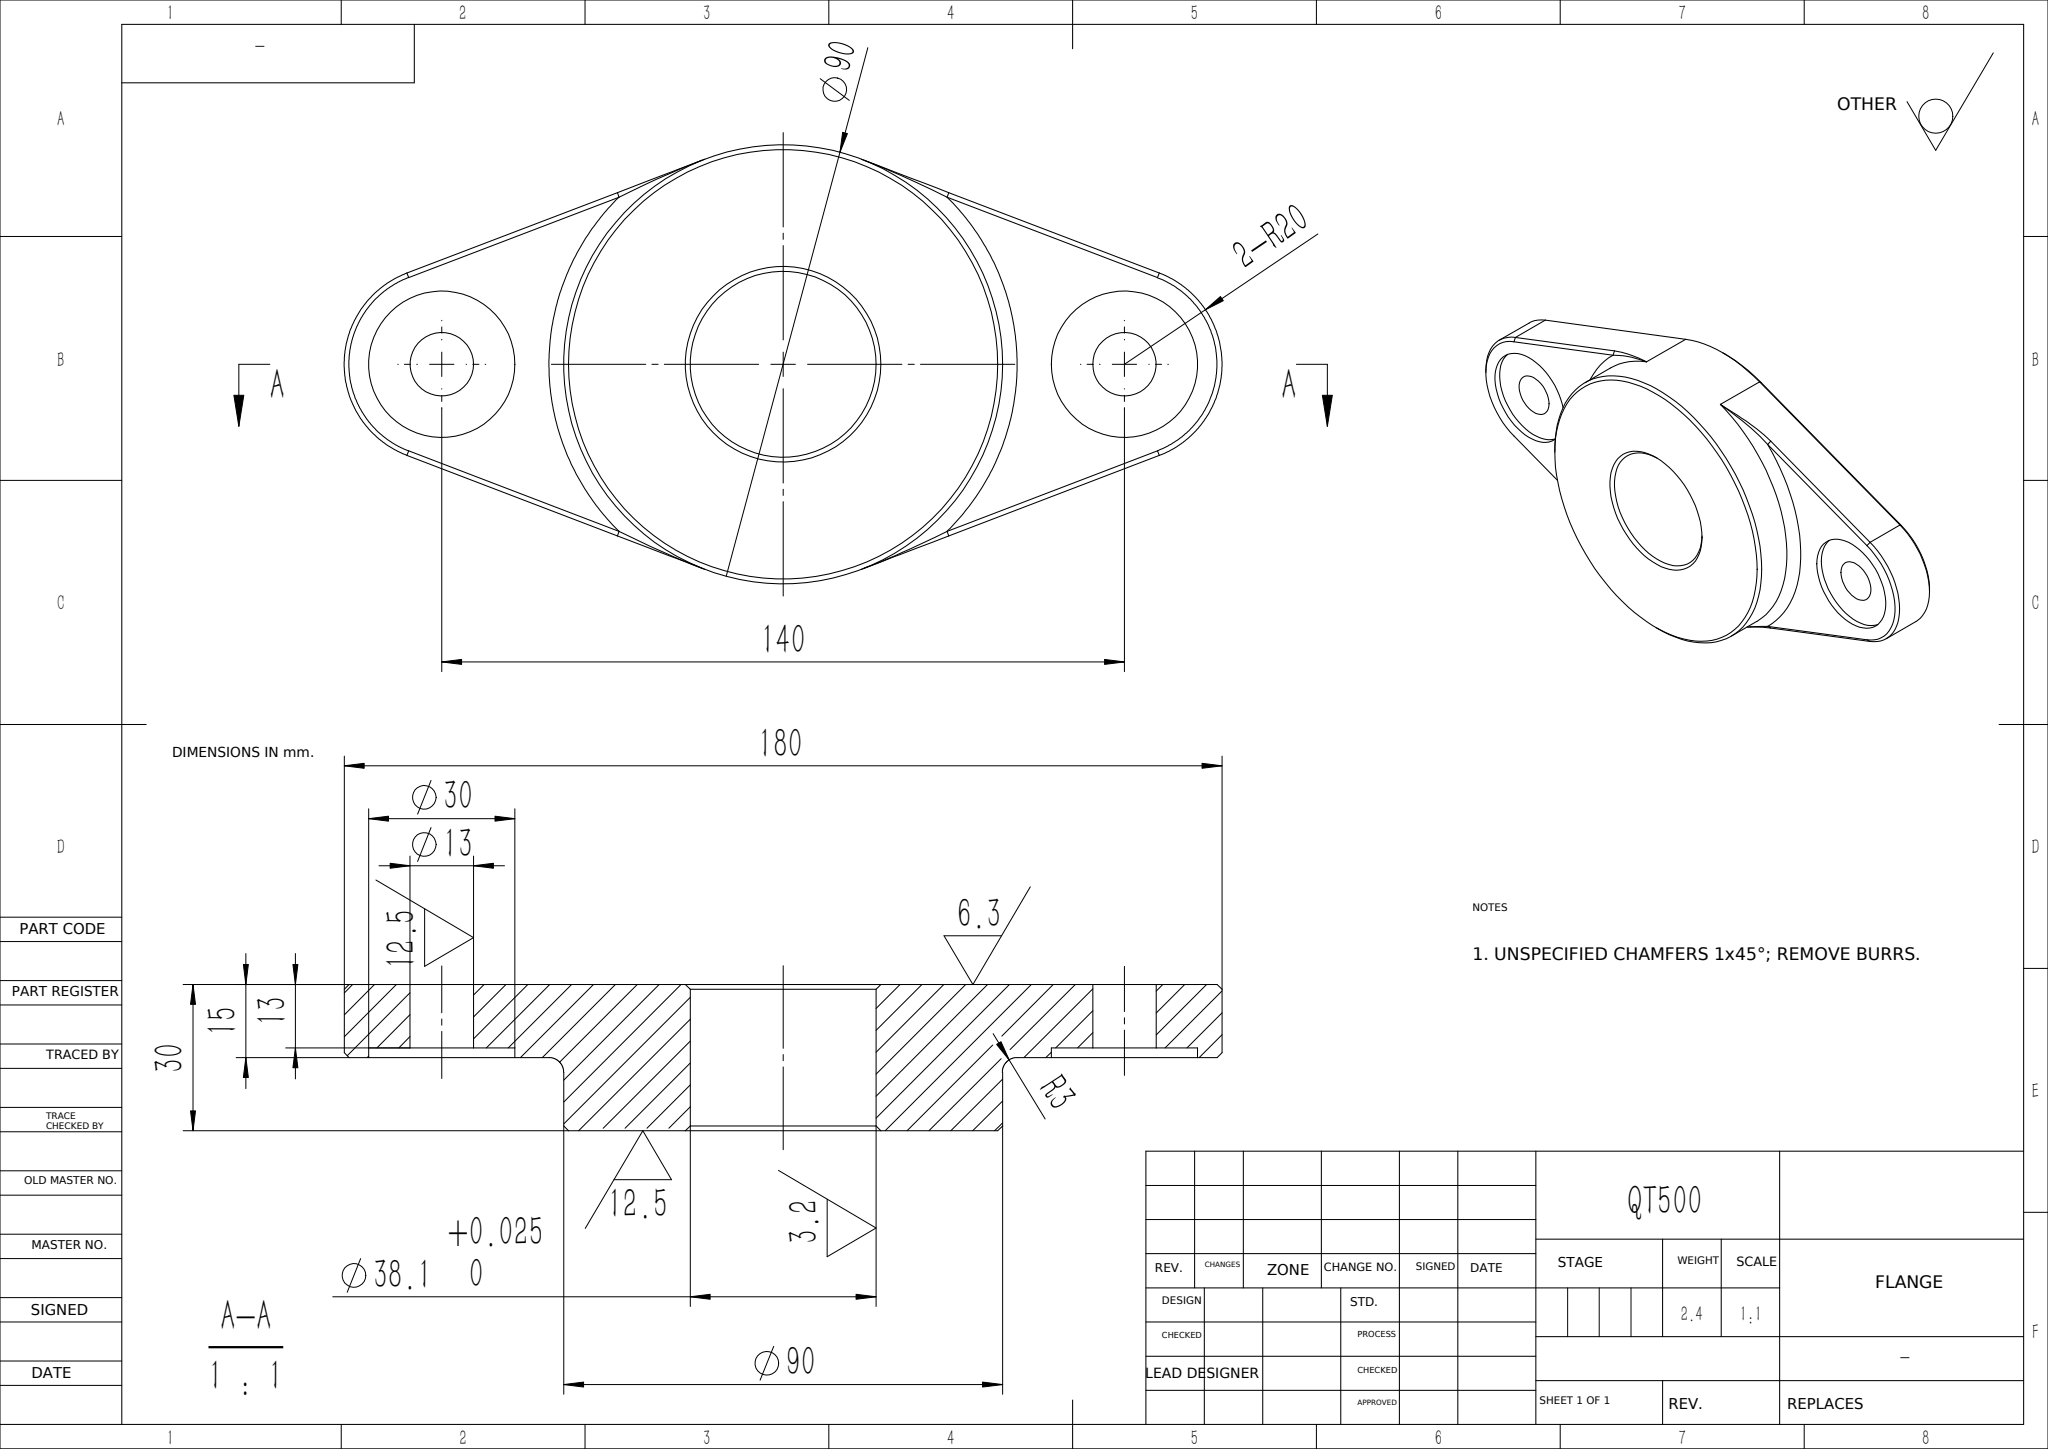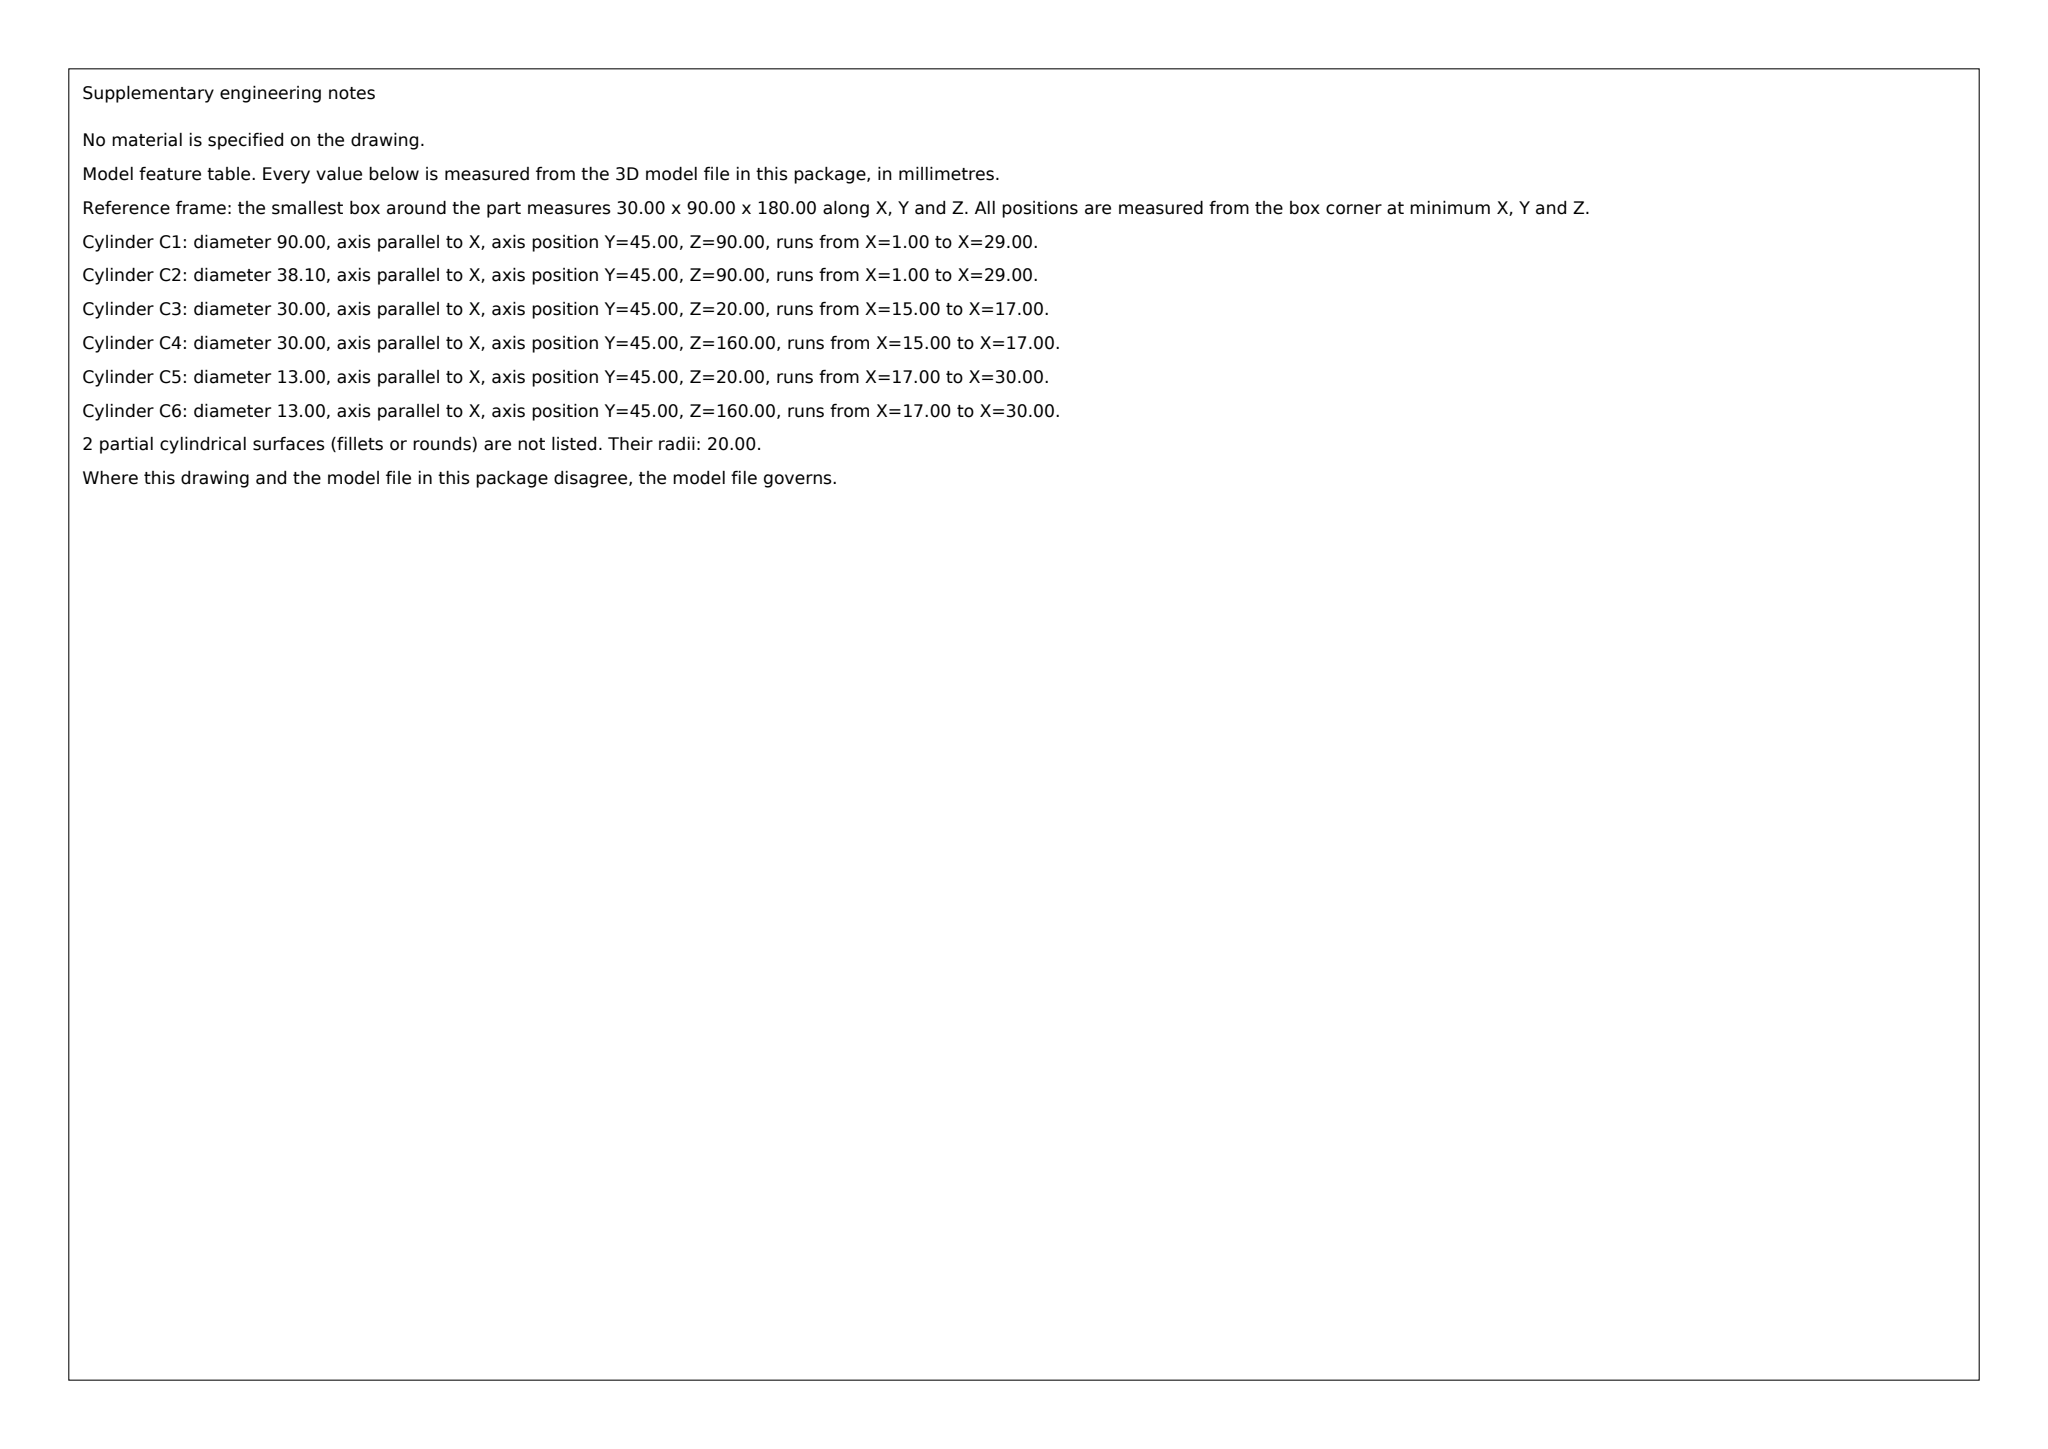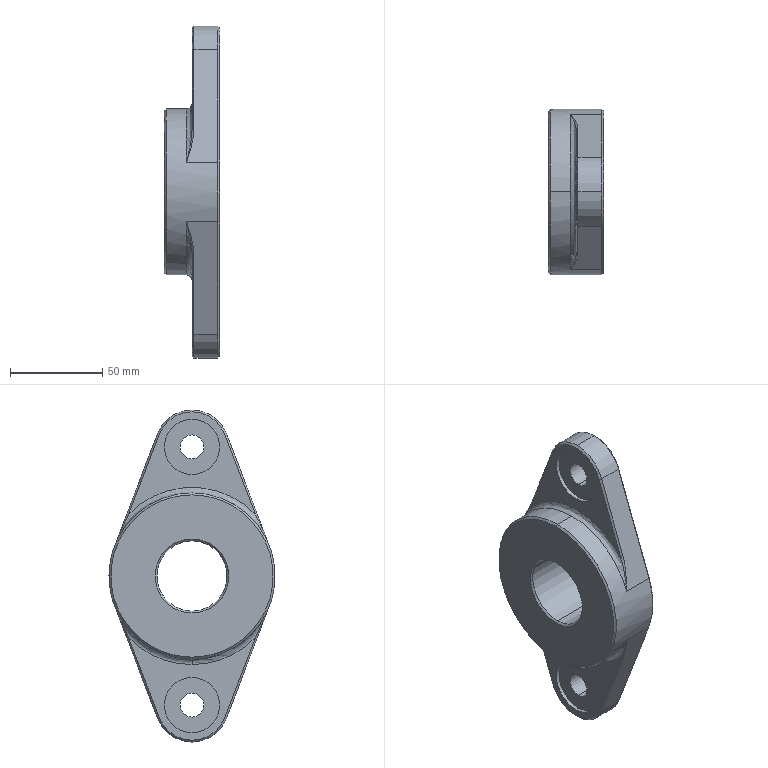Part | SolidWorks | mm | 1 solid | 54 faces | box 30 x 90 x 180 mm | volume 218853 mm3 | plane 18 | cylinder 15 | cone 14 | spline 4 | torus 3 | commonest cylinder face diameters 30 x4 13 x4 40 x3 38.1 x2 90 x2